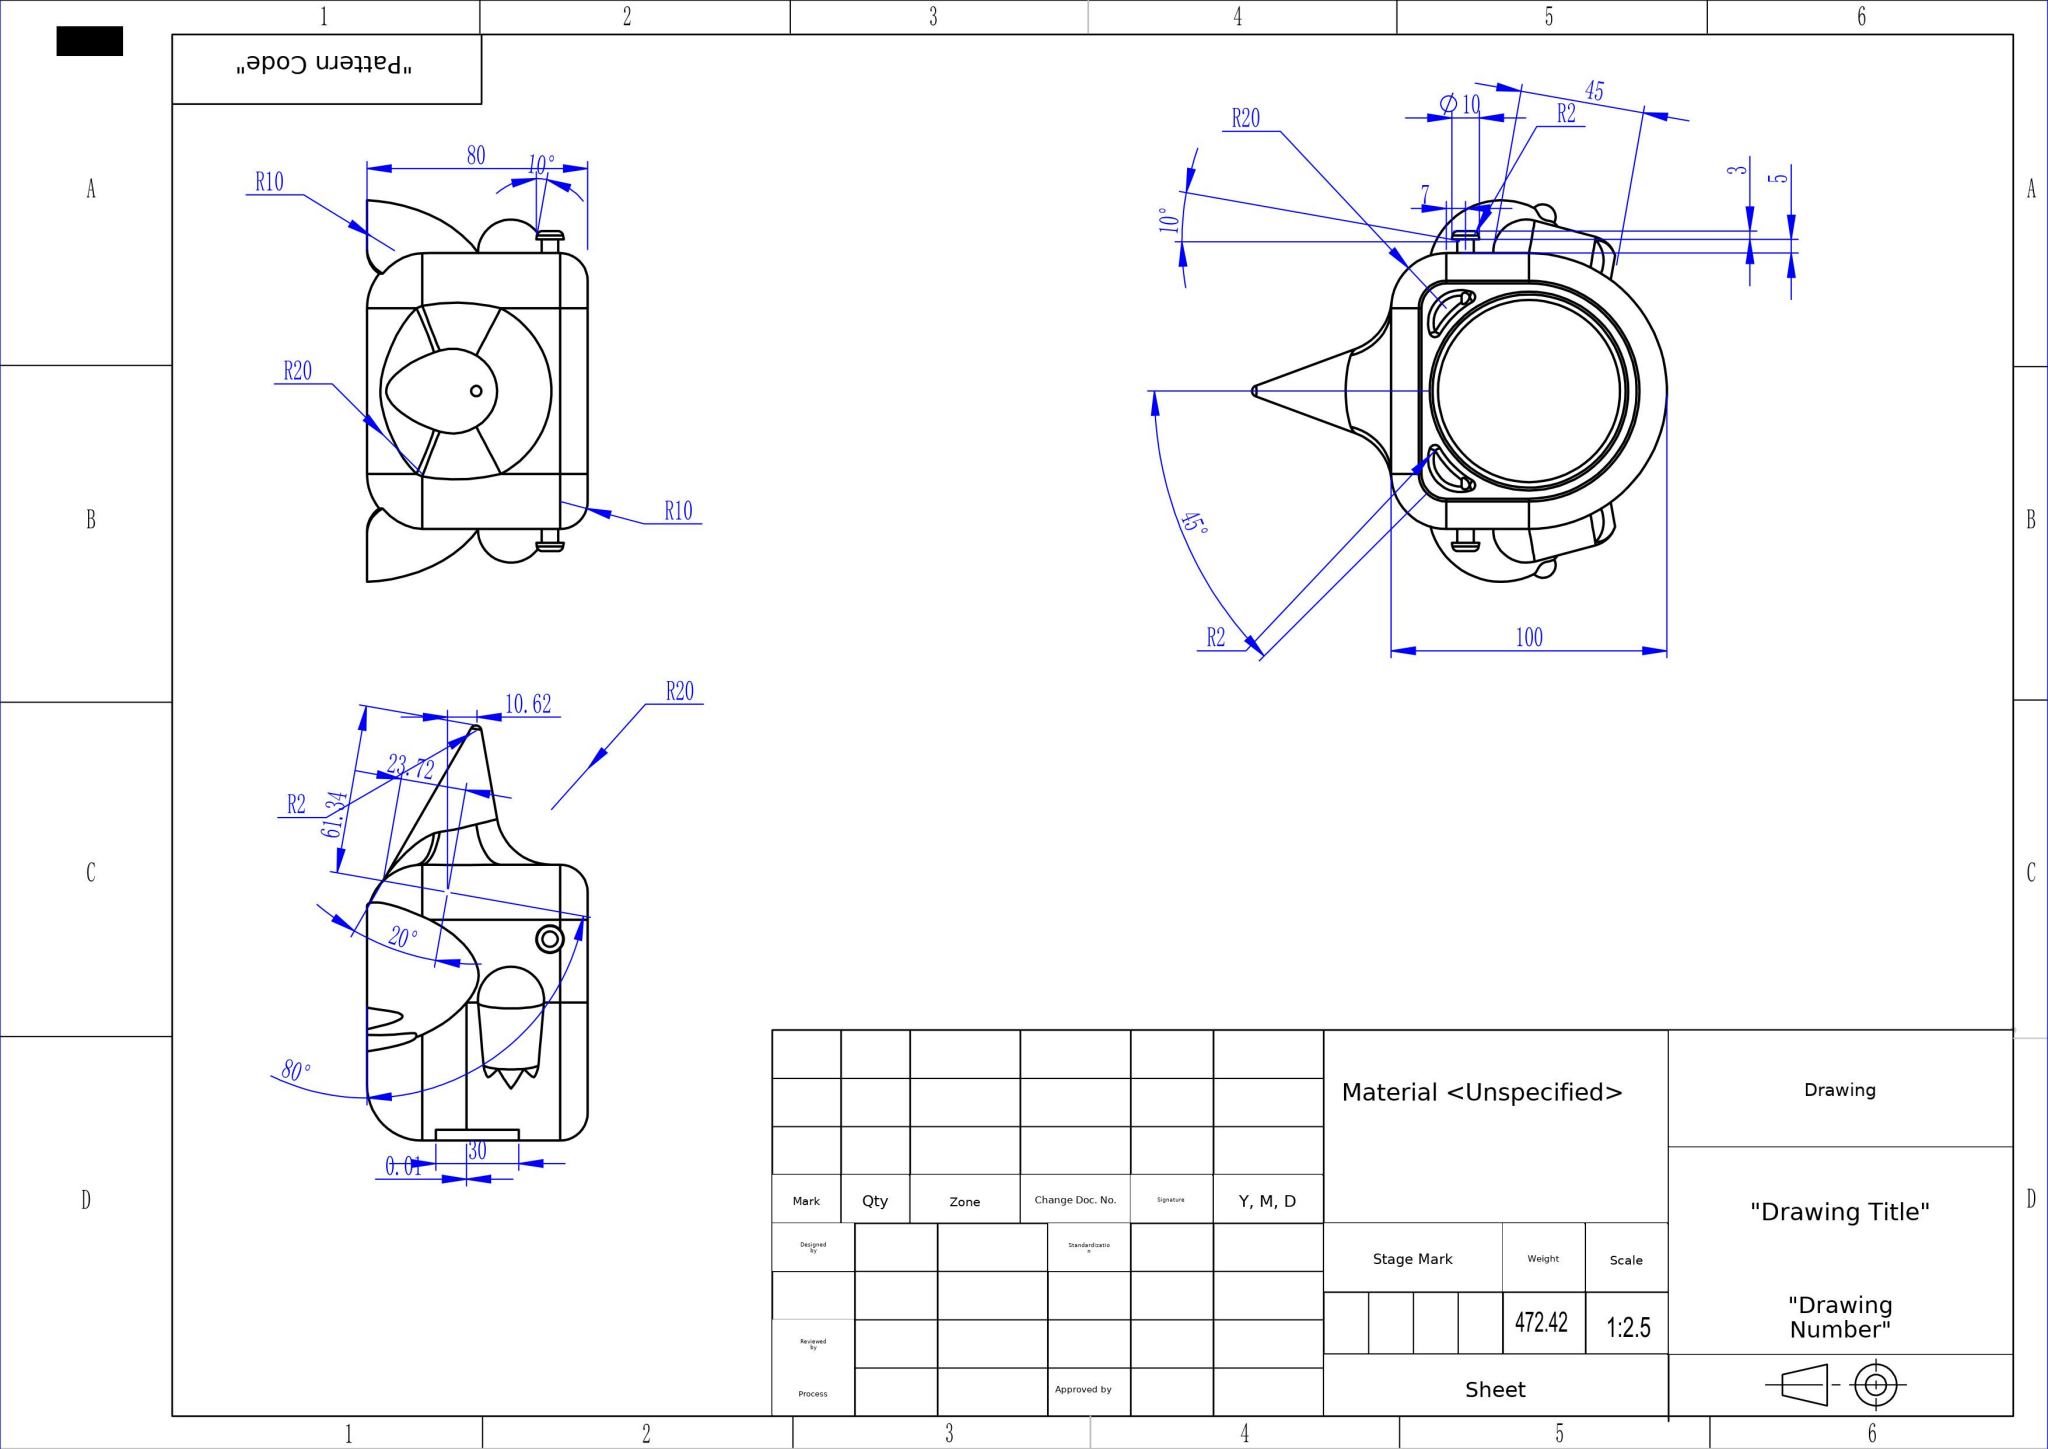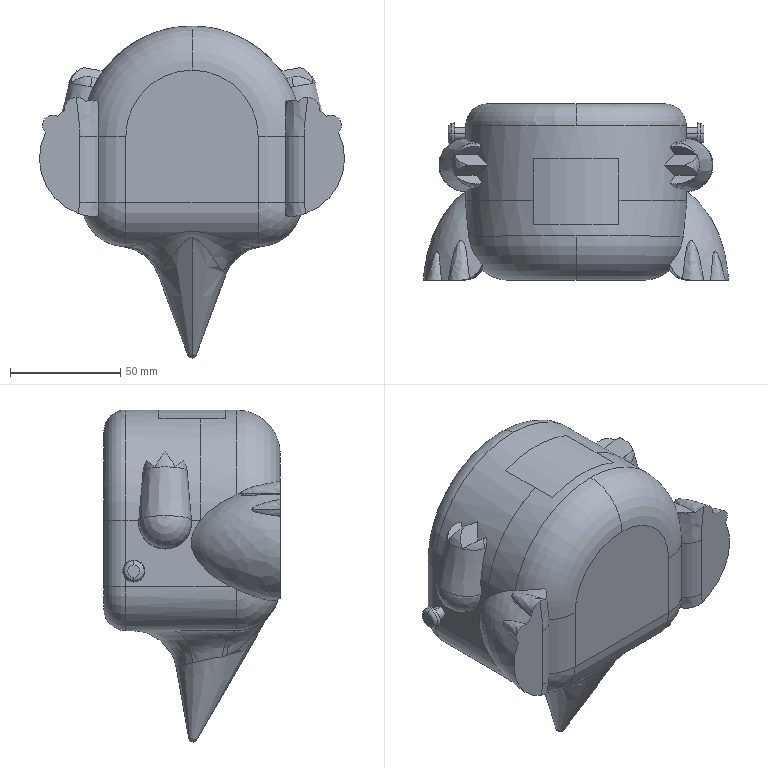Part | SolidWorks | mm | material <Unspecified> | 1 solid | 131 faces | box 138.27 x 80 x 150.46 mm | volume 472431 mm3 | cylinder 31 | plane 27 | sphere 21 | spline 20 | torus 20 | cone 12 | commonest cylinder face diameters 6 x6 4 x6 40 x5 20 x5 100 x3 70 x2 64.287 x2 23.748 x2